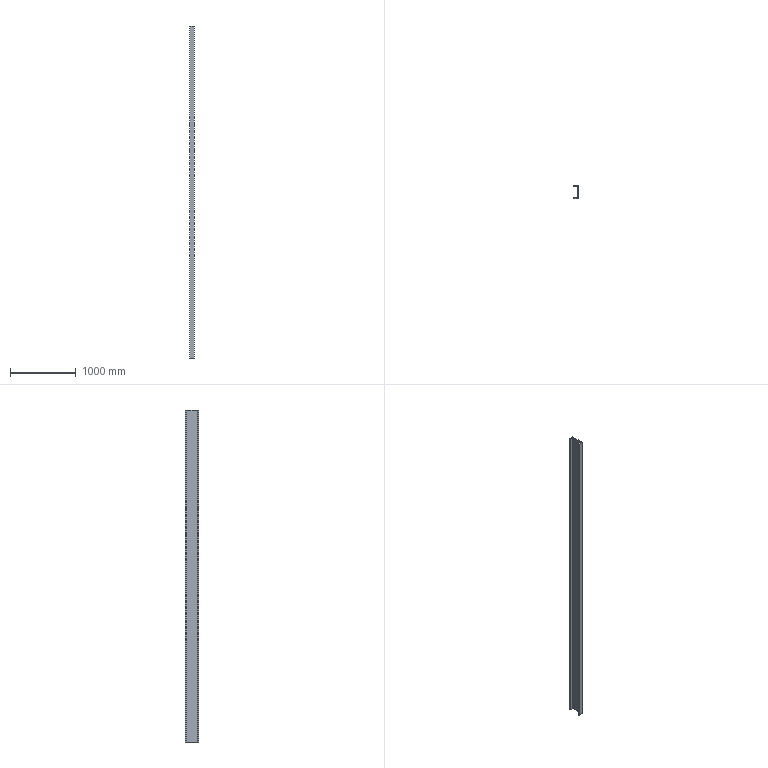Component | SolidWorks | ChannelSteel-1 | 1 solid | 14 faces | box 65 x 200 x 5049 mm | volume 14291166 mm3 | plane 10 | cylinder 4 | commonest cylinder face diameters 10 x2 20 x2
build123d program:
from build123d import *

# Parameters (mm, degrees)
CHANNEL_STEEL_16_1_DEPTH = 5049


with BuildPart() as part:
    # Sketch1 → Channel Steel 16_1 (new body)
    with BuildSketch(Plane.YZ):
        with BuildLine():
            Line((0, 0), (0, -200))
            Line((0, -200), (-65, -200))
            Line((-65, -200), (-65, -196.59))
            ThreePointArc((-65, -196.59), (-63.636, -193.158), (-60.287, -191.598))
            Line((-60.287, -191.598), (-17.926, -189.162))
            ThreePointArc((-17.926, -189.162), (-11.229, -186.043), (-8.5, -179.178))
            Line((-8.5, -179.178), (-8.5, -20.822))
            ThreePointArc((-8.5, -20.822), (-11.229, -13.957), (-17.926, -10.838))
            Line((-17.926, -10.838), (-60.287, -8.402))
            ThreePointArc((-60.287, -8.402), (-63.636, -6.842), (-65, -3.41))
            Line((-65, -3.41), (-65, 0))
            Line((-65, 0), (0, 0))
        make_face()
    extrude(amount=CHANNEL_STEEL_16_1_DEPTH)


solid = part.part

# Placed as in the assembly
solid = solid.moved(Location((1912.304, -594.846, 5213.5), (90, 0, -90)))
STEP:
#1=COLOUR_RGB('',0.7922,0.8196,0.9333);
#2=FILL_AREA_STYLE_COLOUR('',#1);
#3=FILL_AREA_STYLE('',(#2));
#4=SURFACE_STYLE_FILL_AREA(#3);
#5=SURFACE_SIDE_STYLE('',(#4));
#6=SURFACE_STYLE_USAGE(.BOTH.,#5);
#7=PRESENTATION_STYLE_ASSIGNMENT((#6));
#8=CARTESIAN_POINT('',(72.729,-15.545,205.256));
#9=VERTEX_POINT('',#8);
#10=CARTESIAN_POINT('',(75.288,-15.545,205.256));
#11=VERTEX_POINT('',#10);
#12=CARTESIAN_POINT('',(75.288,-15.545,205.256));
#13=DIRECTION('',(1.,-0.,-0.));
#14=VECTOR('',#13,39.37);
#15=LINE('',#12,#14);
#16=EDGE_CURVE('',#9,#11,#15,.T.);
#17=ORIENTED_EDGE('',*,*,#16,.T.);
#18=CARTESIAN_POINT('',(75.288,-15.545,6.476));
#19=VERTEX_POINT('',#18);
#20=CARTESIAN_POINT('',(75.288,-15.545,6.476));
#21=DIRECTION('',(0.,0.,1.));
#22=VECTOR('',#21,39.37);
#23=LINE('',#20,#22);
#24=EDGE_CURVE('',#19,#11,#23,.T.);
#25=ORIENTED_EDGE('',*,*,#24,.F.);
#26=CARTESIAN_POINT('',(72.729,-15.545,6.476));
#27=VERTEX_POINT('',#26);
#28=CARTESIAN_POINT('',(75.288,-15.545,6.476));
#29=DIRECTION('',(1.,-0.,-0.));
#30=VECTOR('',#29,39.37);
#31=LINE('',#28,#30);
#32=EDGE_CURVE('',#27,#19,#31,.T.);
#33=ORIENTED_EDGE('',*,*,#32,.F.);
#34=CARTESIAN_POINT('',(72.729,-15.545,6.476));
#35=DIRECTION('',(0.,0.,1.));
#36=VECTOR('',#35,39.37);
#37=LINE('',#34,#36);
#38=EDGE_CURVE('',#27,#9,#37,.T.);
#39=ORIENTED_EDGE('',*,*,#38,.T.);
#40=EDGE_LOOP('',(#17,#25,#33,#39));
#41=FACE_OUTER_BOUND('',#40,.T.);
#42=CARTESIAN_POINT('',(75.288,-15.545,6.476));
#43=DIRECTION('',(-0.,-1.,0.));
#44=DIRECTION('',(-0.,-0.,-1.));
#45=AXIS2_PLACEMENT_3D('',#42,#43,#44);
#46=PLANE('',#45);
#47=ADVANCED_FACE('',(#41),#46,.F.);
#48=CARTESIAN_POINT('',(75.288,-23.419,205.256));
#49=VERTEX_POINT('',#48);
#50=CARTESIAN_POINT('',(75.288,-23.419,205.256));
#51=DIRECTION('',(-0.,-1.,0.));
#52=VECTOR('',#51,39.37);
#53=LINE('',#50,#52);
#54=EDGE_CURVE('',#11,#49,#53,.T.);
#55=ORIENTED_EDGE('',*,*,#54,.T.);
#56=CARTESIAN_POINT('',(75.288,-23.419,6.476));
#57=VERTEX_POINT('',#56);
#58=CARTESIAN_POINT('',(75.288,-23.419,6.476));
#59=DIRECTION('',(0.,0.,1.));
#60=VECTOR('',#59,39.37);
#61=LINE('',#58,#60);
#62=EDGE_CURVE('',#57,#49,#61,.T.);
#63=ORIENTED_EDGE('',*,*,#62,.F.);
#64=CARTESIAN_POINT('',(75.288,-23.419,6.476));
#65=DIRECTION('',(-0.,-1.,0.));
#66=VECTOR('',#65,39.37);
#67=LINE('',#64,#66);
#68=EDGE_CURVE('',#19,#57,#67,.T.);
#69=ORIENTED_EDGE('',*,*,#68,.F.);
#70=ORIENTED_EDGE('',*,*,#24,.T.);
#71=EDGE_LOOP('',(#55,#63,#69,#70));
#72=FACE_OUTER_BOUND('',#71,.T.);
#73=CARTESIAN_POINT('',(75.288,-23.419,6.476));
#74=DIRECTION('',(-1.,0.,0.));
#75=DIRECTION('',(0.,1.,-0.));
#76=AXIS2_PLACEMENT_3D('',#73,#74,#75);
#77=PLANE('',#76);
#78=ADVANCED_FACE('',(#72),#77,.F.);
#79=CARTESIAN_POINT('',(72.729,-23.419,205.256));
#80=VERTEX_POINT('',#79);
#81=CARTESIAN_POINT('',(75.288,-23.419,205.256));
#82=DIRECTION('',(-1.,0.,0.));
#83=VECTOR('',#82,39.37);
#84=LINE('',#81,#83);
#85=EDGE_CURVE('',#49,#80,#84,.T.);
#86=ORIENTED_EDGE('',*,*,#85,.T.);
#87=CARTESIAN_POINT('',(72.729,-23.419,6.476));
#88=VERTEX_POINT('',#87);
#89=CARTESIAN_POINT('',(72.729,-23.419,6.476));
#90=DIRECTION('',(0.,0.,1.));
#91=VECTOR('',#90,39.37);
#92=LINE('',#89,#91);
#93=EDGE_CURVE('',#88,#80,#92,.T.);
#94=ORIENTED_EDGE('',*,*,#93,.F.);
#95=CARTESIAN_POINT('',(75.288,-23.419,6.476));
#96=DIRECTION('',(-1.,0.,0.));
#97=VECTOR('',#96,39.37);
#98=LINE('',#95,#97);
#99=EDGE_CURVE('',#57,#88,#98,.T.);
#100=ORIENTED_EDGE('',*,*,#99,.F.);
#101=ORIENTED_EDGE('',*,*,#62,.T.);
#102=EDGE_LOOP('',(#86,#94,#100,#101));
#103=FACE_OUTER_BOUND('',#102,.T.);
#104=CARTESIAN_POINT('',(75.288,-23.419,6.476));
#105=DIRECTION('',(0.,1.,-0.));
#106=DIRECTION('',(1.,-0.,-0.));
#107=AXIS2_PLACEMENT_3D('',#104,#105,#106);
#108=PLANE('',#107);
#109=ADVANCED_FACE('',(#103),#108,.F.);
#110=CARTESIAN_POINT('',(72.729,-23.285,205.256));
#111=VERTEX_POINT('',#110);
#112=CARTESIAN_POINT('',(72.729,-23.285,205.256));
#113=DIRECTION('',(0.,1.,-0.));
#114=VECTOR('',#113,39.37);
#115=LINE('',#112,#114);
#116=EDGE_CURVE('',#80,#111,#115,.T.);
#117=ORIENTED_EDGE('',*,*,#116,.T.);
#118=CARTESIAN_POINT('',(72.729,-23.285,6.476));
#119=VERTEX_POINT('',#118);
#120=CARTESIAN_POINT('',(72.729,-23.285,6.476));
#121=DIRECTION('',(0.,0.,1.));
#122=VECTOR('',#121,39.37);
#123=LINE('',#120,#122);
#124=EDGE_CURVE('',#119,#111,#123,.T.);
#125=ORIENTED_EDGE('',*,*,#124,.F.);
#126=CARTESIAN_POINT('',(72.729,-23.285,6.476));
#127=DIRECTION('',(0.,1.,-0.));
#128=VECTOR('',#127,39.37);
#129=LINE('',#126,#128);
#130=EDGE_CURVE('',#88,#119,#129,.T.);
#131=ORIENTED_EDGE('',*,*,#130,.F.);
#132=ORIENTED_EDGE('',*,*,#93,.T.);
#133=EDGE_LOOP('',(#117,#125,#131,#132));
#134=FACE_OUTER_BOUND('',#133,.T.);
#135=CARTESIAN_POINT('',(72.729,-23.285,6.476));
#136=DIRECTION('',(1.,-0.,-0.));
#137=DIRECTION('',(-0.,-1.,0.));
#138=AXIS2_PLACEMENT_3D('',#135,#136,#137);
#139=PLANE('',#138);
#140=ADVANCED_FACE('',(#134),#139,.F.);
#141=CARTESIAN_POINT('',(72.914,-23.088,205.256));
#142=VERTEX_POINT('',#141);
#143=CARTESIAN_POINT('',(72.925,-23.285,205.256));
#144=DIRECTION('',(-0.,-0.,-1.));
#145=DIRECTION('',(0.,1.,0.));
#146=AXIS2_PLACEMENT_3D('',#143,#144,#145);
#147=CIRCLE('',#146,0.1969);
#148=EDGE_CURVE('',#111,#142,#147,.T.);
#149=ORIENTED_EDGE('',*,*,#148,.T.);
#150=CARTESIAN_POINT('',(72.914,-23.088,6.476));
#151=VERTEX_POINT('',#150);
#152=CARTESIAN_POINT('',(72.914,-23.088,6.476));
#153=DIRECTION('',(0.,0.,1.));
#154=VECTOR('',#153,39.37);
#155=LINE('',#152,#154);
#156=EDGE_CURVE('',#151,#142,#155,.T.);
#157=ORIENTED_EDGE('',*,*,#156,.F.);
#158=CARTESIAN_POINT('',(72.925,-23.285,6.476));
#159=DIRECTION('',(-0.,-0.,-1.));
#160=DIRECTION('',(0.,1.,0.));
#161=AXIS2_PLACEMENT_3D('',#158,#159,#160);
#162=CIRCLE('',#161,0.1969);
#163=EDGE_CURVE('',#119,#151,#162,.T.);
#164=ORIENTED_EDGE('',*,*,#163,.F.);
#165=ORIENTED_EDGE('',*,*,#124,.T.);
#166=EDGE_LOOP('',(#149,#157,#164,#165));
#167=FACE_OUTER_BOUND('',#166,.T.);
#168=CARTESIAN_POINT('',(72.925,-23.285,6.476));
#169=DIRECTION('',(0.,0.,1.));
#170=DIRECTION('',(0.,-1.,0.));
#171=AXIS2_PLACEMENT_3D('',#168,#169,#170);
#172=CYLINDRICAL_SURFACE('',#171,0.1969);
#173=ADVANCED_FACE('',(#167),#172,.T.);
#174=CARTESIAN_POINT('',(74.582,-22.992,205.256));
#175=VERTEX_POINT('',#174);
#176=CARTESIAN_POINT('',(74.582,-22.992,205.256));
#177=DIRECTION('',(0.9983,0.05743,-0.));
#178=VECTOR('',#177,39.37);
#179=LINE('',#176,#178);
#180=EDGE_CURVE('',#142,#175,#179,.T.);
#181=ORIENTED_EDGE('',*,*,#180,.T.);
#182=CARTESIAN_POINT('',(74.582,-22.992,6.476));
#183=VERTEX_POINT('',#182);
#184=CARTESIAN_POINT('',(74.582,-22.992,6.476));
#185=DIRECTION('',(0.,0.,1.));
#186=VECTOR('',#185,39.37);
#187=LINE('',#184,#186);
#188=EDGE_CURVE('',#183,#175,#187,.T.);
#189=ORIENTED_EDGE('',*,*,#188,.F.);
#190=CARTESIAN_POINT('',(74.582,-22.992,6.476));
#191=DIRECTION('',(0.9983,0.05743,-0.));
#192=VECTOR('',#191,39.37);
#193=LINE('',#190,#192);
#194=EDGE_CURVE('',#151,#183,#193,.T.);
#195=ORIENTED_EDGE('',*,*,#194,.F.);
#196=ORIENTED_EDGE('',*,*,#156,.T.);
#197=EDGE_LOOP('',(#181,#189,#195,#196));
#198=FACE_OUTER_BOUND('',#197,.T.);
#199=CARTESIAN_POINT('',(74.582,-22.992,6.476));
#200=DIRECTION('',(0.05743,-0.9983,0.));
#201=DIRECTION('',(-0.9983,-0.05743,0.));
#202=AXIS2_PLACEMENT_3D('',#199,#200,#201);
#203=PLANE('',#202);
#204=ADVANCED_FACE('',(#198),#203,.F.);
#205=CARTESIAN_POINT('',(74.953,-22.599,205.256));
#206=VERTEX_POINT('',#205);
#207=CARTESIAN_POINT('',(74.559,-22.599,205.256));
#208=DIRECTION('',(0.,0.,1.));
#209=DIRECTION('',(0.,-1.,0.));
#210=AXIS2_PLACEMENT_3D('',#207,#208,#209);
#211=CIRCLE('',#210,0.3937);
#212=EDGE_CURVE('',#175,#206,#211,.T.);
#213=ORIENTED_EDGE('',*,*,#212,.T.);
#214=CARTESIAN_POINT('',(74.953,-22.599,6.476));
#215=VERTEX_POINT('',#214);
#216=CARTESIAN_POINT('',(74.953,-22.599,6.476));
#217=DIRECTION('',(0.,0.,1.));
#218=VECTOR('',#217,39.37);
#219=LINE('',#216,#218);
#220=EDGE_CURVE('',#215,#206,#219,.T.);
#221=ORIENTED_EDGE('',*,*,#220,.F.);
#222=CARTESIAN_POINT('',(74.559,-22.599,6.476));
#223=DIRECTION('',(0.,0.,1.));
#224=DIRECTION('',(0.,-1.,0.));
#225=AXIS2_PLACEMENT_3D('',#222,#223,#224);
#226=CIRCLE('',#225,0.3937);
#227=EDGE_CURVE('',#183,#215,#226,.T.);
#228=ORIENTED_EDGE('',*,*,#227,.F.);
#229=ORIENTED_EDGE('',*,*,#188,.T.);
#230=EDGE_LOOP('',(#213,#221,#228,#229));
#231=FACE_OUTER_BOUND('',#230,.T.);
#232=CARTESIAN_POINT('',(74.559,-22.599,6.476));
#233=DIRECTION('',(0.,0.,1.));
#234=DIRECTION('',(0.,-1.,0.));
#235=AXIS2_PLACEMENT_3D('',#232,#233,#234);
#236=CYLINDRICAL_SURFACE('',#235,0.3937);
#237=ADVANCED_FACE('',(#231),#236,.F.);
#238=CARTESIAN_POINT('',(74.953,-16.365,205.256));
#239=VERTEX_POINT('',#238);
#240=CARTESIAN_POINT('',(74.953,-16.365,205.256));
#241=DIRECTION('',(0.,1.,-0.));
#242=VECTOR('',#241,39.37);
#243=LINE('',#240,#242);
#244=EDGE_CURVE('',#206,#239,#243,.T.);
#245=ORIENTED_EDGE('',*,*,#244,.T.);
#246=CARTESIAN_POINT('',(74.953,-16.365,6.476));
#247=VERTEX_POINT('',#246);
#248=CARTESIAN_POINT('',(74.953,-16.365,6.476));
#249=DIRECTION('',(0.,0.,1.));
#250=VECTOR('',#249,39.37);
#251=LINE('',#248,#250);
#252=EDGE_CURVE('',#247,#239,#251,.T.);
#253=ORIENTED_EDGE('',*,*,#252,.F.);
#254=CARTESIAN_POINT('',(74.953,-16.365,6.476));
#255=DIRECTION('',(0.,1.,-0.));
#256=VECTOR('',#255,39.37);
#257=LINE('',#254,#256);
#258=EDGE_CURVE('',#215,#247,#257,.T.);
#259=ORIENTED_EDGE('',*,*,#258,.F.);
#260=ORIENTED_EDGE('',*,*,#220,.T.);
#261=EDGE_LOOP('',(#245,#253,#259,#260));
#262=FACE_OUTER_BOUND('',#261,.T.);
#263=CARTESIAN_POINT('',(74.953,-16.365,6.476));
#264=DIRECTION('',(1.,-0.,-0.));
#265=DIRECTION('',(-0.,-1.,0.));
#266=AXIS2_PLACEMENT_3D('',#263,#264,#265);
#267=PLANE('',#266);
#268=ADVANCED_FACE('',(#262),#267,.F.);
#269=CARTESIAN_POINT('',(74.582,-15.972,205.256));
#270=VERTEX_POINT('',#269);
#271=CARTESIAN_POINT('',(74.559,-16.365,205.256));
#272=DIRECTION('',(0.,0.,1.));
#273=DIRECTION('',(0.,-1.,0.));
#274=AXIS2_PLACEMENT_3D('',#271,#272,#273);
#275=CIRCLE('',#274,0.3937);
#276=EDGE_CURVE('',#239,#270,#275,.T.);
#277=ORIENTED_EDGE('',*,*,#276,.T.);
#278=CARTESIAN_POINT('',(74.582,-15.972,6.476));
#279=VERTEX_POINT('',#278);
#280=CARTESIAN_POINT('',(74.582,-15.972,6.476));
#281=DIRECTION('',(0.,0.,1.));
#282=VECTOR('',#281,39.37);
#283=LINE('',#280,#282);
#284=EDGE_CURVE('',#279,#270,#283,.T.);
#285=ORIENTED_EDGE('',*,*,#284,.F.);
#286=CARTESIAN_POINT('',(74.559,-16.365,6.476));
#287=DIRECTION('',(0.,0.,1.));
#288=DIRECTION('',(0.,-1.,0.));
#289=AXIS2_PLACEMENT_3D('',#286,#287,#288);
#290=CIRCLE('',#289,0.3937);
#291=EDGE_CURVE('',#247,#279,#290,.T.);
#292=ORIENTED_EDGE('',*,*,#291,.F.);
#293=ORIENTED_EDGE('',*,*,#252,.T.);
#294=EDGE_LOOP('',(#277,#285,#292,#293));
#295=FACE_OUTER_BOUND('',#294,.T.);
#296=CARTESIAN_POINT('',(74.559,-16.365,6.476));
#297=DIRECTION('',(0.,0.,1.));
#298=DIRECTION('',(0.,-1.,0.));
#299=AXIS2_PLACEMENT_3D('',#296,#297,#298);
#300=CYLINDRICAL_SURFACE('',#299,0.3937);
#301=ADVANCED_FACE('',(#295),#300,.F.);
#302=CARTESIAN_POINT('',(72.914,-15.876,205.256));
#303=VERTEX_POINT('',#302);
#304=CARTESIAN_POINT('',(74.582,-15.972,205.256));
#305=DIRECTION('',(-0.9983,0.05743,0.));
#306=VECTOR('',#305,39.37);
#307=LINE('',#304,#306);
#308=EDGE_CURVE('',#270,#303,#307,.T.);
#309=ORIENTED_EDGE('',*,*,#308,.T.);
#310=CARTESIAN_POINT('',(72.914,-15.876,6.476));
#311=VERTEX_POINT('',#310);
#312=CARTESIAN_POINT('',(72.914,-15.876,6.476));
#313=DIRECTION('',(0.,0.,1.));
#314=VECTOR('',#313,39.37);
#315=LINE('',#312,#314);
#316=EDGE_CURVE('',#311,#303,#315,.T.);
#317=ORIENTED_EDGE('',*,*,#316,.F.);
#318=CARTESIAN_POINT('',(74.582,-15.972,6.476));
#319=DIRECTION('',(-0.9983,0.05743,0.));
#320=VECTOR('',#319,39.37);
#321=LINE('',#318,#320);
#322=EDGE_CURVE('',#279,#311,#321,.T.);
#323=ORIENTED_EDGE('',*,*,#322,.F.);
#324=ORIENTED_EDGE('',*,*,#284,.T.);
#325=EDGE_LOOP('',(#309,#317,#323,#324));
#326=FACE_OUTER_BOUND('',#325,.T.);
#327=CARTESIAN_POINT('',(74.582,-15.972,6.476));
#328=DIRECTION('',(0.05743,0.9983,-0.));
#329=DIRECTION('',(0.9983,-0.05743,-0.));
#330=AXIS2_PLACEMENT_3D('',#327,#328,#329);
#331=PLANE('',#330);
#332=ADVANCED_FACE('',(#326),#331,.F.);
#333=CARTESIAN_POINT('',(72.729,-15.679,205.256));
#334=VERTEX_POINT('',#333);
#335=CARTESIAN_POINT('',(72.925,-15.679,205.256));
#336=DIRECTION('',(-0.,-0.,-1.));
#337=DIRECTION('',(0.,1.,0.));
#338=AXIS2_PLACEMENT_3D('',#335,#336,#337);
#339=CIRCLE('',#338,0.1969);
#340=EDGE_CURVE('',#303,#334,#339,.T.);
#341=ORIENTED_EDGE('',*,*,#340,.T.);
#342=CARTESIAN_POINT('',(72.729,-15.679,6.476));
#343=VERTEX_POINT('',#342);
#344=CARTESIAN_POINT('',(72.729,-15.679,6.476));
#345=DIRECTION('',(0.,0.,1.));
#346=VECTOR('',#345,39.37);
#347=LINE('',#344,#346);
#348=EDGE_CURVE('',#343,#334,#347,.T.);
#349=ORIENTED_EDGE('',*,*,#348,.F.);
#350=CARTESIAN_POINT('',(72.925,-15.679,6.476));
#351=DIRECTION('',(-0.,-0.,-1.));
#352=DIRECTION('',(0.,1.,0.));
#353=AXIS2_PLACEMENT_3D('',#350,#351,#352);
#354=CIRCLE('',#353,0.1969);
#355=EDGE_CURVE('',#311,#343,#354,.T.);
#356=ORIENTED_EDGE('',*,*,#355,.F.);
#357=ORIENTED_EDGE('',*,*,#316,.T.);
#358=EDGE_LOOP('',(#341,#349,#356,#357));
#359=FACE_OUTER_BOUND('',#358,.T.);
#360=CARTESIAN_POINT('',(72.925,-15.679,6.476));
#361=DIRECTION('',(0.,0.,1.));
#362=DIRECTION('',(0.,-1.,0.));
#363=AXIS2_PLACEMENT_3D('',#360,#361,#362);
#364=CYLINDRICAL_SURFACE('',#363,0.1969);
#365=ADVANCED_FACE('',(#359),#364,.T.);
#366=CARTESIAN_POINT('',(72.729,-15.679,205.256));
#367=DIRECTION('',(-0.,1.,-0.));
#368=VECTOR('',#367,39.37);
#369=LINE('',#366,#368);
#370=EDGE_CURVE('',#334,#9,#369,.T.);
#371=ORIENTED_EDGE('',*,*,#370,.T.);
#372=ORIENTED_EDGE('',*,*,#38,.F.);
#373=CARTESIAN_POINT('',(72.729,-15.679,6.476));
#374=DIRECTION('',(-0.,1.,-0.));
#375=VECTOR('',#374,39.37);
#376=LINE('',#373,#375);
#377=EDGE_CURVE('',#343,#27,#376,.T.);
#378=ORIENTED_EDGE('',*,*,#377,.F.);
#379=ORIENTED_EDGE('',*,*,#348,.T.);
#380=EDGE_LOOP('',(#371,#372,#378,#379));
#381=FACE_OUTER_BOUND('',#380,.T.);
#382=CARTESIAN_POINT('',(72.729,-15.679,6.476));
#383=DIRECTION('',(1.,0.,-0.));
#384=DIRECTION('',(0.,-1.,0.));
#385=AXIS2_PLACEMENT_3D('',#382,#383,#384);
#386=PLANE('',#385);
#387=ADVANCED_FACE('',(#381),#386,.F.);
#388=ORIENTED_EDGE('',*,*,#32,.T.);
#389=ORIENTED_EDGE('',*,*,#68,.T.);
#390=ORIENTED_EDGE('',*,*,#99,.T.);
#391=ORIENTED_EDGE('',*,*,#130,.T.);
#392=ORIENTED_EDGE('',*,*,#163,.T.);
#393=ORIENTED_EDGE('',*,*,#194,.T.);
#394=ORIENTED_EDGE('',*,*,#227,.T.);
#395=ORIENTED_EDGE('',*,*,#258,.T.);
#396=ORIENTED_EDGE('',*,*,#291,.T.);
#397=ORIENTED_EDGE('',*,*,#322,.T.);
#398=ORIENTED_EDGE('',*,*,#355,.T.);
#399=ORIENTED_EDGE('',*,*,#377,.T.);
#400=EDGE_LOOP('',(#388,#389,#390,#391,#392,#393,#394,#395,#396,#397,#398,#399));
#401=FACE_OUTER_BOUND('',#400,.T.);
#402=CARTESIAN_POINT('',(72.925,-15.679,6.476));
#403=DIRECTION('',(-0.,-0.,-1.));
#404=DIRECTION('',(0.,1.,-0.));
#405=AXIS2_PLACEMENT_3D('',#402,#403,#404);
#406=PLANE('',#405);
#407=ADVANCED_FACE('',(#401),#406,.T.);
#408=ORIENTED_EDGE('',*,*,#16,.F.);
#409=ORIENTED_EDGE('',*,*,#370,.F.);
#410=ORIENTED_EDGE('',*,*,#340,.F.);
#411=ORIENTED_EDGE('',*,*,#308,.F.);
#412=ORIENTED_EDGE('',*,*,#276,.F.);
#413=ORIENTED_EDGE('',*,*,#244,.F.);
#414=ORIENTED_EDGE('',*,*,#212,.F.);
#415=ORIENTED_EDGE('',*,*,#180,.F.);
#416=ORIENTED_EDGE('',*,*,#148,.F.);
#417=ORIENTED_EDGE('',*,*,#116,.F.);
#418=ORIENTED_EDGE('',*,*,#85,.F.);
#419=ORIENTED_EDGE('',*,*,#54,.F.);
#420=EDGE_LOOP('',(#408,#409,#410,#411,#412,#413,#414,#415,#416,#417,#418,#419));
#421=FACE_OUTER_BOUND('',#420,.T.);
#422=CARTESIAN_POINT('',(72.925,-15.679,205.256));
#423=DIRECTION('',(-0.,-0.,-1.));
#424=DIRECTION('',(0.,1.,-0.));
#425=AXIS2_PLACEMENT_3D('',#422,#423,#424);
#426=PLANE('',#425);
#427=ADVANCED_FACE('',(#421),#426,.F.);
#428=CLOSED_SHELL('',(#47,#78,#109,#140,#173,#204,#237,#268,#301,#332,#365,#387,#407,#427));
#429=MANIFOLD_SOLID_BREP('',#428);
#430=STYLED_ITEM('',(#7),#429);
#431=PRESENTATION_LAYER_ASSIGNMENT('','',(#430));
#432=(LENGTH_UNIT()NAMED_UNIT(*)SI_UNIT($,.METRE.));
#433=LENGTH_MEASURE_WITH_UNIT(LENGTH_MEASURE(0.0254),#432);
#434=DIMENSIONAL_EXPONENTS(1.,0.,0.,0.,0.,0.,0.);
#435=(CONVERSION_BASED_UNIT('',#433)LENGTH_UNIT()NAMED_UNIT(#434));
#436=UNCERTAINTY_MEASURE_WITH_UNIT(LENGTH_MEASURE(0.00001),#435,'','');
#437=(NAMED_UNIT(*)PLANE_ANGLE_UNIT()SI_UNIT($,.RADIAN.));
#438=(NAMED_UNIT(*)SI_UNIT($,.STERADIAN.)SOLID_ANGLE_UNIT());
#439=(GEOMETRIC_REPRESENTATION_CONTEXT(3)GLOBAL_UNCERTAINTY_ASSIGNED_CONTEXT((#436))GLOBAL_UNIT_ASSIGNED_CONTEXT((#435,#437,#438))REPRESENTATION_CONTEXT('',''));
#440=MECHANICAL_DESIGN_GEOMETRIC_PRESENTATION_REPRESENTATION('',(#430),#439);
#441=CARTESIAN_POINT('',(0.,0.,0.));
#442=DIRECTION('',(0.,0.,1.));
#443=DIRECTION('',(1.,0.,0.));
#444=AXIS2_PLACEMENT_3D('',#441,#442,#443);
#445=(LENGTH_UNIT()NAMED_UNIT(*)SI_UNIT($,.METRE.));
#446=LENGTH_MEASURE_WITH_UNIT(LENGTH_MEASURE(0.0254),#445);
#447=DIMENSIONAL_EXPONENTS(1.,0.,0.,0.,0.,0.,0.);
#448=(CONVERSION_BASED_UNIT('',#446)LENGTH_UNIT()NAMED_UNIT(#447));
#449=UNCERTAINTY_MEASURE_WITH_UNIT(LENGTH_MEASURE(0.00001),#448,'','');
#450=(NAMED_UNIT(*)PLANE_ANGLE_UNIT()SI_UNIT($,.RADIAN.));
#451=(NAMED_UNIT(*)SI_UNIT($,.STERADIAN.)SOLID_ANGLE_UNIT());
#452=(GEOMETRIC_REPRESENTATION_CONTEXT(3)GLOBAL_UNCERTAINTY_ASSIGNED_CONTEXT((#449))GLOBAL_UNIT_ASSIGNED_CONTEXT((#448,#450,#451))REPRESENTATION_CONTEXT('',''));
#453=ADVANCED_BREP_SHAPE_REPRESENTATION('',(#429,#444),#452);